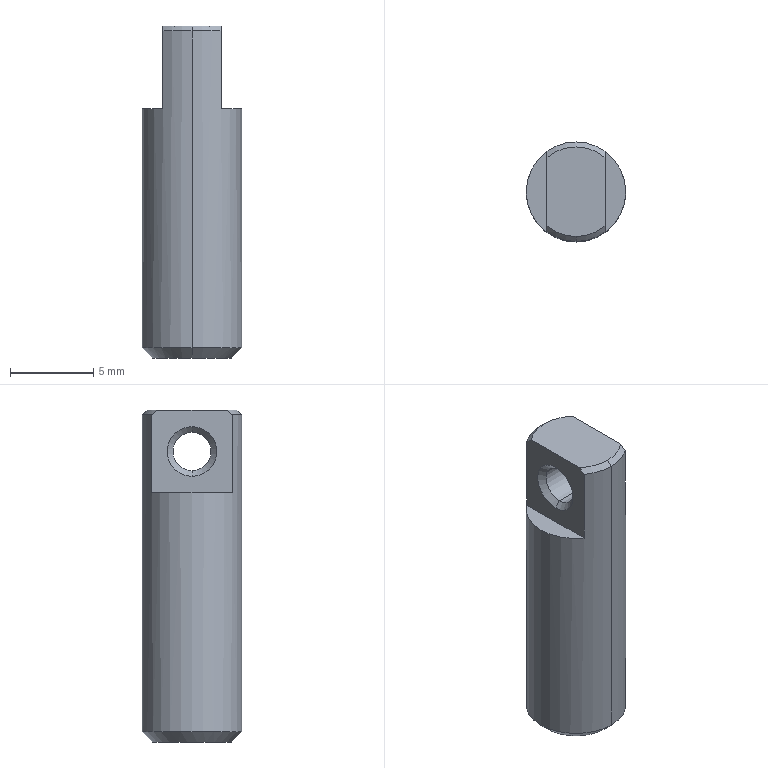Component | SolidWorks | SpringPillarFFE01-D6-L20-1 | 1 solid | 19 faces | box 6 x 6 x 20 mm | volume 504 mm3 | cone 9 | plane 6 | cylinder 4 | commonest cylinder face diameters 6 x2 2.3 x2 | material Purchased Part
STEP:
#1=CARTESIAN_POINT('',(-2.126,-0.315,-0.6845));
#2=VERTEX_POINT('',#1);
#3=CARTESIAN_POINT('',(-2.126,-0.5512,-0.6845));
#4=VERTEX_POINT('',#3);
#5=CARTESIAN_POINT('',(-2.126,-0.4331,-0.6845));
#6=DIRECTION('',(0.,0.,1.));
#7=DIRECTION('',(0.,1.,0.));
#8=AXIS2_PLACEMENT_3D('',#5,#6,#7);
#9=CIRCLE('',#8,0.1181);
#10=EDGE_CURVE('',#2,#4,#9,.T.);
#11=ORIENTED_EDGE('',*,*,#10,.T.);
#12=CARTESIAN_POINT('',(-2.126,-0.5512,0.06693));
#13=VERTEX_POINT('',#12);
#14=CARTESIAN_POINT('',(-2.126,-0.5512,-0.7087));
#15=DIRECTION('',(0.,0.,1.));
#16=VECTOR('',#15,39.37);
#17=LINE('',#14,#16);
#18=EDGE_CURVE('',#4,#13,#17,.T.);
#19=ORIENTED_EDGE('',*,*,#18,.T.);
#20=CARTESIAN_POINT('',(-2.195,-0.529,0.06693));
#21=VERTEX_POINT('',#20);
#22=CARTESIAN_POINT('',(-2.126,-0.4331,0.06693));
#23=DIRECTION('',(0.,0.,-1.));
#24=DIRECTION('',(0.,1.,0.));
#25=AXIS2_PLACEMENT_3D('',#22,#23,#24);
#26=CIRCLE('',#25,0.1181);
#27=EDGE_CURVE('',#13,#21,#26,.T.);
#28=ORIENTED_EDGE('',*,*,#27,.T.);
#29=CARTESIAN_POINT('',(-2.195,-0.529,-0.1181));
#30=VERTEX_POINT('',#29);
#31=CARTESIAN_POINT('',(-2.195,-0.529,-0.7087));
#32=DIRECTION('',(0.,0.,-1.));
#33=VECTOR('',#32,39.37);
#34=LINE('',#31,#33);
#35=EDGE_CURVE('',#21,#30,#34,.T.);
#36=ORIENTED_EDGE('',*,*,#35,.T.);
#37=CARTESIAN_POINT('',(-2.195,-0.3371,-0.1181));
#38=VERTEX_POINT('',#37);
#39=CARTESIAN_POINT('',(-2.126,-0.4331,-0.1181));
#40=DIRECTION('',(0.,0.,-1.));
#41=DIRECTION('',(0.,1.,0.));
#42=AXIS2_PLACEMENT_3D('',#39,#40,#41);
#43=CIRCLE('',#42,0.1181);
#44=EDGE_CURVE('',#30,#38,#43,.T.);
#45=ORIENTED_EDGE('',*,*,#44,.T.);
#46=CARTESIAN_POINT('',(-2.195,-0.3371,0.06693));
#47=VERTEX_POINT('',#46);
#48=CARTESIAN_POINT('',(-2.195,-0.3371,-0.7087));
#49=DIRECTION('',(0.,0.,1.));
#50=VECTOR('',#49,39.37);
#51=LINE('',#48,#50);
#52=EDGE_CURVE('',#38,#47,#51,.T.);
#53=ORIENTED_EDGE('',*,*,#52,.T.);
#54=CARTESIAN_POINT('',(-2.126,-0.315,0.06693));
#55=VERTEX_POINT('',#54);
#56=CARTESIAN_POINT('',(-2.126,-0.4331,0.06693));
#57=DIRECTION('',(0.,0.,-1.));
#58=DIRECTION('',(-0.,1.,0.));
#59=AXIS2_PLACEMENT_3D('',#56,#57,#58);
#60=CIRCLE('',#59,0.1181);
#61=EDGE_CURVE('',#47,#55,#60,.T.);
#62=ORIENTED_EDGE('',*,*,#61,.T.);
#63=CARTESIAN_POINT('',(-2.126,-0.315,-0.7087));
#64=DIRECTION('',(0.,0.,1.));
#65=VECTOR('',#64,39.37);
#66=LINE('',#63,#65);
#67=EDGE_CURVE('',#2,#55,#66,.T.);
#68=ORIENTED_EDGE('',*,*,#67,.F.);
#69=EDGE_LOOP('',(#11,#19,#28,#36,#45,#53,#62,#68));
#70=FACE_OUTER_BOUND('',#69,.T.);
#71=CARTESIAN_POINT('',(-2.126,-0.4331,-0.7087));
#72=DIRECTION('',(0.,0.,1.));
#73=DIRECTION('',(0.,1.,0.));
#74=AXIS2_PLACEMENT_3D('',#71,#72,#73);
#75=CYLINDRICAL_SURFACE('',#74,0.1181);
#76=ADVANCED_FACE('',(#70),#75,.T.);
#77=CARTESIAN_POINT('',(-2.057,-0.514,0.07874));
#78=VERTEX_POINT('',#77);
#79=CARTESIAN_POINT('',(-2.126,-0.5394,0.07874));
#80=VERTEX_POINT('',#79);
#81=CARTESIAN_POINT('',(-2.126,-0.4331,0.07874));
#82=DIRECTION('',(0.,0.,-1.));
#83=DIRECTION('',(0.,-1.,0.));
#84=AXIS2_PLACEMENT_3D('',#81,#82,#83);
#85=CIRCLE('',#84,0.1063);
#86=EDGE_CURVE('',#78,#80,#85,.T.);
#87=ORIENTED_EDGE('',*,*,#86,.T.);
#88=CARTESIAN_POINT('',(-2.126,-0.5512,0.06693));
#89=DIRECTION('',(0.,-0.7071,-0.7071));
#90=VECTOR('',#89,39.37);
#91=LINE('',#88,#90);
#92=EDGE_CURVE('',#80,#13,#91,.T.);
#93=ORIENTED_EDGE('',*,*,#92,.T.);
#94=CARTESIAN_POINT('',(-2.057,-0.529,0.06693));
#95=VERTEX_POINT('',#94);
#96=CARTESIAN_POINT('',(-2.126,-0.4331,0.06693));
#97=DIRECTION('',(0.,0.,-1.));
#98=DIRECTION('',(0.,1.,0.));
#99=AXIS2_PLACEMENT_3D('',#96,#97,#98);
#100=CIRCLE('',#99,0.1181);
#101=EDGE_CURVE('',#95,#13,#100,.T.);
#102=ORIENTED_EDGE('',*,*,#101,.F.);
#103=CARTESIAN_POINT('',(-2.057,-0.514,0.07874));
#104=CARTESIAN_POINT('',(-2.057,-0.5191,0.07489));
#105=CARTESIAN_POINT('',(-2.057,-0.5241,0.07094));
#106=CARTESIAN_POINT('',(-2.057,-0.529,0.06693));
#107=B_SPLINE_CURVE_WITH_KNOTS('',3,(#103,#104,#105,#106),.UNSPECIFIED.,.F.,.F.,(4,4),(0.,0.0004846),.UNSPECIFIED.);
#108=EDGE_CURVE('',#78,#95,#107,.T.);
#109=ORIENTED_EDGE('',*,*,#108,.F.);
#110=EDGE_LOOP('',(#87,#93,#102,#109));
#111=FACE_OUTER_BOUND('',#110,.T.);
#112=CARTESIAN_POINT('',(-2.126,-0.4331,0.06693));
#113=DIRECTION('',(0.,0.,-1.));
#114=DIRECTION('',(0.,-1.,0.));
#115=AXIS2_PLACEMENT_3D('',#112,#113,#114);
#116=CONICAL_SURFACE('',#115,0.1181,0.7854);
#117=ADVANCED_FACE('',(#111),#116,.T.);
#118=CARTESIAN_POINT('',(-2.126,-0.3391,-0.7087));
#119=VERTEX_POINT('',#118);
#120=CARTESIAN_POINT('',(-2.126,-0.527,-0.7087));
#121=VERTEX_POINT('',#120);
#122=CARTESIAN_POINT('',(-2.126,-0.4331,-0.7087));
#123=DIRECTION('',(0.,0.,1.));
#124=DIRECTION('',(0.,1.,0.));
#125=AXIS2_PLACEMENT_3D('',#122,#123,#124);
#126=CIRCLE('',#125,0.09396);
#127=EDGE_CURVE('',#119,#121,#126,.T.);
#128=ORIENTED_EDGE('',*,*,#127,.T.);
#129=CARTESIAN_POINT('',(-2.126,-0.5512,-0.6845));
#130=DIRECTION('',(-0.,-0.7071,0.7071));
#131=VECTOR('',#130,39.37);
#132=LINE('',#129,#131);
#133=EDGE_CURVE('',#121,#4,#132,.T.);
#134=ORIENTED_EDGE('',*,*,#133,.T.);
#135=ORIENTED_EDGE('',*,*,#10,.F.);
#136=CARTESIAN_POINT('',(-2.126,-0.315,-0.6845));
#137=DIRECTION('',(0.,0.7071,0.7071));
#138=VECTOR('',#137,39.37);
#139=LINE('',#136,#138);
#140=EDGE_CURVE('',#119,#2,#139,.T.);
#141=ORIENTED_EDGE('',*,*,#140,.F.);
#142=EDGE_LOOP('',(#128,#134,#135,#141));
#143=FACE_OUTER_BOUND('',#142,.T.);
#144=CARTESIAN_POINT('',(-2.126,-0.4331,-0.6845));
#145=DIRECTION('',(0.,0.,1.));
#146=DIRECTION('',(0.,1.,0.));
#147=AXIS2_PLACEMENT_3D('',#144,#145,#146);
#148=CONICAL_SURFACE('',#147,0.1181,0.7854);
#149=ADVANCED_FACE('',(#143),#148,.T.);
#150=CARTESIAN_POINT('',(-2.071,-0.4331,0.02559));
#151=VERTEX_POINT('',#150);
#152=CARTESIAN_POINT('',(-2.071,-0.4331,-0.06496));
#153=VERTEX_POINT('',#152);
#154=CARTESIAN_POINT('',(-2.071,-0.4331,-0.01969));
#155=DIRECTION('',(1.,0.,0.));
#156=DIRECTION('',(0.,0.,-1.));
#157=AXIS2_PLACEMENT_3D('',#154,#155,#156);
#158=CIRCLE('',#157,0.04528);
#159=EDGE_CURVE('',#151,#153,#158,.T.);
#160=ORIENTED_EDGE('',*,*,#159,.F.);
#161=CARTESIAN_POINT('',(-2.057,-0.4331,0.03937));
#162=VERTEX_POINT('',#161);
#163=CARTESIAN_POINT('',(-2.057,-0.4331,0.03937));
#164=DIRECTION('',(0.7071,0.,0.7071));
#165=VECTOR('',#164,39.37);
#166=LINE('',#163,#165);
#167=EDGE_CURVE('',#151,#162,#166,.T.);
#168=ORIENTED_EDGE('',*,*,#167,.T.);
#169=CARTESIAN_POINT('',(-2.057,-0.4331,-0.07874));
#170=VERTEX_POINT('',#169);
#171=CARTESIAN_POINT('',(-2.057,-0.4331,-0.01969));
#172=DIRECTION('',(-1.,0.,0.));
#173=DIRECTION('',(0.,0.,-1.));
#174=AXIS2_PLACEMENT_3D('',#171,#172,#173);
#175=CIRCLE('',#174,0.05906);
#176=EDGE_CURVE('',#170,#162,#175,.T.);
#177=ORIENTED_EDGE('',*,*,#176,.F.);
#178=CARTESIAN_POINT('',(-2.057,-0.4331,-0.07874));
#179=DIRECTION('',(0.7071,0.,-0.7071));
#180=VECTOR('',#179,39.37);
#181=LINE('',#178,#180);
#182=EDGE_CURVE('',#153,#170,#181,.T.);
#183=ORIENTED_EDGE('',*,*,#182,.F.);
#184=EDGE_LOOP('',(#160,#168,#177,#183));
#185=FACE_OUTER_BOUND('',#184,.T.);
#186=CARTESIAN_POINT('',(-2.057,-0.4331,-0.01969));
#187=DIRECTION('',(1.,0.,0.));
#188=DIRECTION('',(0.,0.,-1.));
#189=AXIS2_PLACEMENT_3D('',#186,#187,#188);
#190=CONICAL_SURFACE('',#189,0.05906,0.7854);
#191=ADVANCED_FACE('',(#185),#190,.F.);
#192=CARTESIAN_POINT('',(-2.181,-0.4331,-0.06496));
#193=VERTEX_POINT('',#192);
#194=CARTESIAN_POINT('',(-2.181,-0.4331,0.02559));
#195=VERTEX_POINT('',#194);
#196=CARTESIAN_POINT('',(-2.181,-0.4331,-0.01969));
#197=DIRECTION('',(-1.,0.,0.));
#198=DIRECTION('',(0.,0.,1.));
#199=AXIS2_PLACEMENT_3D('',#196,#197,#198);
#200=CIRCLE('',#199,0.04528);
#201=EDGE_CURVE('',#193,#195,#200,.T.);
#202=ORIENTED_EDGE('',*,*,#201,.F.);
#203=CARTESIAN_POINT('',(-2.195,-0.4331,-0.07874));
#204=VERTEX_POINT('',#203);
#205=CARTESIAN_POINT('',(-2.195,-0.4331,-0.07874));
#206=DIRECTION('',(-0.7071,0.,-0.7071));
#207=VECTOR('',#206,39.37);
#208=LINE('',#205,#207);
#209=EDGE_CURVE('',#193,#204,#208,.T.);
#210=ORIENTED_EDGE('',*,*,#209,.T.);
#211=CARTESIAN_POINT('',(-2.195,-0.4331,0.03937));
#212=VERTEX_POINT('',#211);
#213=CARTESIAN_POINT('',(-2.195,-0.4331,-0.01969));
#214=DIRECTION('',(1.,0.,0.));
#215=DIRECTION('',(0.,0.,1.));
#216=AXIS2_PLACEMENT_3D('',#213,#214,#215);
#217=CIRCLE('',#216,0.05906);
#218=EDGE_CURVE('',#212,#204,#217,.T.);
#219=ORIENTED_EDGE('',*,*,#218,.F.);
#220=CARTESIAN_POINT('',(-2.195,-0.4331,0.03937));
#221=DIRECTION('',(-0.7071,0.,0.7071));
#222=VECTOR('',#221,39.37);
#223=LINE('',#220,#222);
#224=EDGE_CURVE('',#195,#212,#223,.T.);
#225=ORIENTED_EDGE('',*,*,#224,.F.);
#226=EDGE_LOOP('',(#202,#210,#219,#225));
#227=FACE_OUTER_BOUND('',#226,.T.);
#228=CARTESIAN_POINT('',(-2.195,-0.4331,-0.01969));
#229=DIRECTION('',(-1.,0.,0.));
#230=DIRECTION('',(0.,0.,1.));
#231=AXIS2_PLACEMENT_3D('',#228,#229,#230);
#232=CONICAL_SURFACE('',#231,0.05906,0.7854);
#233=ADVANCED_FACE('',(#227),#232,.F.);
#234=ORIENTED_EDGE('',*,*,#159,.T.);
#235=CARTESIAN_POINT('',(-2.057,-0.4331,-0.06496));
#236=DIRECTION('',(-1.,0.,0.));
#237=VECTOR('',#236,39.37);
#238=LINE('',#235,#237);
#239=EDGE_CURVE('',#153,#193,#238,.T.);
#240=ORIENTED_EDGE('',*,*,#239,.T.);
#241=ORIENTED_EDGE('',*,*,#201,.T.);
#242=CARTESIAN_POINT('',(-2.057,-0.4331,0.02559));
#243=DIRECTION('',(-1.,0.,0.));
#244=VECTOR('',#243,39.37);
#245=LINE('',#242,#244);
#246=EDGE_CURVE('',#151,#195,#245,.T.);
#247=ORIENTED_EDGE('',*,*,#246,.F.);
#248=EDGE_LOOP('',(#234,#240,#241,#247));
#249=FACE_OUTER_BOUND('',#248,.T.);
#250=CARTESIAN_POINT('',(-2.057,-0.4331,-0.01969));
#251=DIRECTION('',(-1.,0.,0.));
#252=DIRECTION('',(0.,0.,1.));
#253=AXIS2_PLACEMENT_3D('',#250,#251,#252);
#254=CYLINDRICAL_SURFACE('',#253,0.04528);
#255=ADVANCED_FACE('',(#249),#254,.F.);
#256=ORIENTED_EDGE('',*,*,#18,.F.);
#257=CARTESIAN_POINT('',(-2.126,-0.4331,-0.6845));
#258=DIRECTION('',(0.,0.,1.));
#259=DIRECTION('',(0.,1.,0.));
#260=AXIS2_PLACEMENT_3D('',#257,#258,#259);
#261=CIRCLE('',#260,0.1181);
#262=EDGE_CURVE('',#4,#2,#261,.T.);
#263=ORIENTED_EDGE('',*,*,#262,.T.);
#264=ORIENTED_EDGE('',*,*,#67,.T.);
#265=CARTESIAN_POINT('',(-2.057,-0.3371,0.06693));
#266=VERTEX_POINT('',#265);
#267=CARTESIAN_POINT('',(-2.126,-0.4331,0.06693));
#268=DIRECTION('',(0.,0.,-1.));
#269=DIRECTION('',(0.,1.,0.));
#270=AXIS2_PLACEMENT_3D('',#267,#268,#269);
#271=CIRCLE('',#270,0.1181);
#272=EDGE_CURVE('',#55,#266,#271,.T.);
#273=ORIENTED_EDGE('',*,*,#272,.T.);
#274=CARTESIAN_POINT('',(-2.057,-0.3371,-0.1181));
#275=VERTEX_POINT('',#274);
#276=CARTESIAN_POINT('',(-2.057,-0.3371,-0.7087));
#277=DIRECTION('',(0.,0.,-1.));
#278=VECTOR('',#277,39.37);
#279=LINE('',#276,#278);
#280=EDGE_CURVE('',#266,#275,#279,.T.);
#281=ORIENTED_EDGE('',*,*,#280,.T.);
#282=CARTESIAN_POINT('',(-2.057,-0.529,-0.1181));
#283=VERTEX_POINT('',#282);
#284=CARTESIAN_POINT('',(-2.126,-0.4331,-0.1181));
#285=DIRECTION('',(0.,0.,-1.));
#286=DIRECTION('',(0.,1.,0.));
#287=AXIS2_PLACEMENT_3D('',#284,#285,#286);
#288=CIRCLE('',#287,0.1181);
#289=EDGE_CURVE('',#275,#283,#288,.T.);
#290=ORIENTED_EDGE('',*,*,#289,.T.);
#291=CARTESIAN_POINT('',(-2.057,-0.529,-0.7087));
#292=DIRECTION('',(0.,0.,1.));
#293=VECTOR('',#292,39.37);
#294=LINE('',#291,#293);
#295=EDGE_CURVE('',#283,#95,#294,.T.);
#296=ORIENTED_EDGE('',*,*,#295,.T.);
#297=ORIENTED_EDGE('',*,*,#101,.T.);
#298=EDGE_LOOP('',(#256,#263,#264,#273,#281,#290,#296,#297));
#299=FACE_OUTER_BOUND('',#298,.T.);
#300=CARTESIAN_POINT('',(-2.126,-0.4331,-0.7087));
#301=DIRECTION('',(0.,0.,1.));
#302=DIRECTION('',(0.,1.,0.));
#303=AXIS2_PLACEMENT_3D('',#300,#301,#302);
#304=CYLINDRICAL_SURFACE('',#303,0.1181);
#305=ADVANCED_FACE('',(#299),#304,.T.);
#306=CARTESIAN_POINT('',(-2.057,-0.315,-0.1181));
#307=DIRECTION('',(0.,-1.,0.));
#308=VECTOR('',#307,39.37);
#309=LINE('',#306,#308);
#310=EDGE_CURVE('',#275,#283,#309,.T.);
#311=ORIENTED_EDGE('',*,*,#310,.T.);
#312=ORIENTED_EDGE('',*,*,#289,.F.);
#313=EDGE_LOOP('',(#311,#312));
#314=FACE_OUTER_BOUND('',#313,.T.);
#315=CARTESIAN_POINT('',(-2.008,-0.315,-0.1181));
#316=DIRECTION('',(0.,0.,1.));
#317=DIRECTION('',(0.,1.,0.));
#318=AXIS2_PLACEMENT_3D('',#315,#316,#317);
#319=PLANE('',#318);
#320=ADVANCED_FACE('',(#314),#319,.T.);
#321=ORIENTED_EDGE('',*,*,#176,.T.);
#322=CARTESIAN_POINT('',(-2.057,-0.4331,-0.01969));
#323=DIRECTION('',(-1.,0.,0.));
#324=DIRECTION('',(0.,0.,-1.));
#325=AXIS2_PLACEMENT_3D('',#322,#323,#324);
#326=CIRCLE('',#325,0.05906);
#327=EDGE_CURVE('',#162,#170,#326,.T.);
#328=ORIENTED_EDGE('',*,*,#327,.T.);
#329=EDGE_LOOP('',(#321,#328));
#330=FACE_BOUND('',#329,.T.);
#331=CARTESIAN_POINT('',(-2.057,-0.3521,0.07874));
#332=VERTEX_POINT('',#331);
#333=CARTESIAN_POINT('',(-2.057,-0.3371,0.06693));
#334=CARTESIAN_POINT('',(-2.057,-0.3421,0.07094));
#335=CARTESIAN_POINT('',(-2.057,-0.3471,0.07489));
#336=CARTESIAN_POINT('',(-2.057,-0.3521,0.07874));
#337=B_SPLINE_CURVE_WITH_KNOTS('',3,(#333,#334,#335,#336),.UNSPECIFIED.,.F.,.F.,(4,4),(0.,0.0004846),.UNSPECIFIED.);
#338=EDGE_CURVE('',#266,#332,#337,.T.);
#339=ORIENTED_EDGE('',*,*,#338,.T.);
#340=CARTESIAN_POINT('',(-2.057,-0.315,0.07874));
#341=DIRECTION('',(0.,-1.,0.));
#342=VECTOR('',#341,39.37);
#343=LINE('',#340,#342);
#344=EDGE_CURVE('',#332,#78,#343,.T.);
#345=ORIENTED_EDGE('',*,*,#344,.T.);
#346=ORIENTED_EDGE('',*,*,#108,.T.);
#347=ORIENTED_EDGE('',*,*,#295,.F.);
#348=ORIENTED_EDGE('',*,*,#310,.F.);
#349=ORIENTED_EDGE('',*,*,#280,.F.);
#350=EDGE_LOOP('',(#339,#345,#346,#347,#348,#349));
#351=FACE_OUTER_BOUND('',#350,.T.);
#352=CARTESIAN_POINT('',(-2.057,-0.315,-0.1181));
#353=DIRECTION('',(1.,0.,0.));
#354=DIRECTION('',(0.,0.,-1.));
#355=AXIS2_PLACEMENT_3D('',#352,#353,#354);
#356=PLANE('',#355);
#357=ADVANCED_FACE('',(#330,#351),#356,.T.);
#358=CARTESIAN_POINT('',(-2.195,-0.3521,0.07874));
#359=VERTEX_POINT('',#358);
#360=CARTESIAN_POINT('',(-2.195,-0.3371,0.06693));
#361=CARTESIAN_POINT('',(-2.195,-0.3421,0.07094));
#362=CARTESIAN_POINT('',(-2.195,-0.3471,0.07489));
#363=CARTESIAN_POINT('',(-2.195,-0.3521,0.07874));
#364=B_SPLINE_CURVE_WITH_KNOTS('',3,(#360,#361,#362,#363),.UNSPECIFIED.,.F.,.F.,(4,4),(0.,0.0004846),.UNSPECIFIED.);
#365=EDGE_CURVE('',#47,#359,#364,.T.);
#366=ORIENTED_EDGE('',*,*,#365,.T.);
#367=CARTESIAN_POINT('',(-2.126,-0.4331,0.07874));
#368=DIRECTION('',(0.,0.,-1.));
#369=DIRECTION('',(0.,-1.,0.));
#370=AXIS2_PLACEMENT_3D('',#367,#368,#369);
#371=CIRCLE('',#370,0.1063);
#372=EDGE_CURVE('',#359,#332,#371,.T.);
#373=ORIENTED_EDGE('',*,*,#372,.T.);
#374=ORIENTED_EDGE('',*,*,#338,.F.);
#375=ORIENTED_EDGE('',*,*,#272,.F.);
#376=ORIENTED_EDGE('',*,*,#61,.F.);
#377=EDGE_LOOP('',(#366,#373,#374,#375,#376));
#378=FACE_OUTER_BOUND('',#377,.T.);
#379=CARTESIAN_POINT('',(-2.126,-0.4331,0.06693));
#380=DIRECTION('',(0.,0.,-1.));
#381=DIRECTION('',(0.,-1.,0.));
#382=AXIS2_PLACEMENT_3D('',#379,#380,#381);
#383=CONICAL_SURFACE('',#382,0.1181,0.7854);
#384=ADVANCED_FACE('',(#378),#383,.T.);
#385=ORIENTED_EDGE('',*,*,#218,.T.);
#386=CARTESIAN_POINT('',(-2.195,-0.4331,-0.01969));
#387=DIRECTION('',(1.,0.,0.));
#388=DIRECTION('',(0.,0.,1.));
#389=AXIS2_PLACEMENT_3D('',#386,#387,#388);
#390=CIRCLE('',#389,0.05906);
#391=EDGE_CURVE('',#204,#212,#390,.T.);
#392=ORIENTED_EDGE('',*,*,#391,.T.);
#393=EDGE_LOOP('',(#385,#392));
#394=FACE_BOUND('',#393,.T.);
#395=CARTESIAN_POINT('',(-2.195,-0.514,0.07874));
#396=VERTEX_POINT('',#395);
#397=CARTESIAN_POINT('',(-2.195,-0.529,0.06693));
#398=CARTESIAN_POINT('',(-2.195,-0.5241,0.07094));
#399=CARTESIAN_POINT('',(-2.195,-0.5191,0.07489));
#400=CARTESIAN_POINT('',(-2.195,-0.514,0.07874));
#401=B_SPLINE_CURVE_WITH_KNOTS('',3,(#397,#398,#399,#400),.UNSPECIFIED.,.F.,.F.,(4,4),(0.,0.0004846),.UNSPECIFIED.);
#402=EDGE_CURVE('',#21,#396,#401,.T.);
#403=ORIENTED_EDGE('',*,*,#402,.T.);
#404=CARTESIAN_POINT('',(-2.195,-0.315,0.07874));
#405=DIRECTION('',(0.,1.,0.));
#406=VECTOR('',#405,39.37);
#407=LINE('',#404,#406);
#408=EDGE_CURVE('',#396,#359,#407,.T.);
#409=ORIENTED_EDGE('',*,*,#408,.T.);
#410=ORIENTED_EDGE('',*,*,#365,.F.);
#411=ORIENTED_EDGE('',*,*,#52,.F.);
#412=CARTESIAN_POINT('',(-2.195,-0.315,-0.1181));
#413=DIRECTION('',(0.,-1.,0.));
#414=VECTOR('',#413,39.37);
#415=LINE('',#412,#414);
#416=EDGE_CURVE('',#38,#30,#415,.T.);
#417=ORIENTED_EDGE('',*,*,#416,.T.);
#418=ORIENTED_EDGE('',*,*,#35,.F.);
#419=EDGE_LOOP('',(#403,#409,#410,#411,#417,#418));
#420=FACE_OUTER_BOUND('',#419,.T.);
#421=CARTESIAN_POINT('',(-2.195,-0.315,0.07874));
#422=DIRECTION('',(-1.,0.,0.));
#423=DIRECTION('',(0.,0.,1.));
#424=AXIS2_PLACEMENT_3D('',#421,#422,#423);
#425=PLANE('',#424);
#426=ADVANCED_FACE('',(#394,#420),#425,.T.);
#427=ORIENTED_EDGE('',*,*,#416,.F.);
#428=ORIENTED_EDGE('',*,*,#44,.F.);
#429=EDGE_LOOP('',(#427,#428));
#430=FACE_OUTER_BOUND('',#429,.T.);
#431=CARTESIAN_POINT('',(-2.195,-0.315,-0.1181));
#432=DIRECTION('',(0.,0.,1.));
#433=DIRECTION('',(0.,1.,0.));
#434=AXIS2_PLACEMENT_3D('',#431,#432,#433);
#435=PLANE('',#434);
#436=ADVANCED_FACE('',(#430),#435,.T.);
#437=ORIENTED_EDGE('',*,*,#92,.F.);
#438=CARTESIAN_POINT('',(-2.126,-0.4331,0.07874));
#439=DIRECTION('',(0.,0.,-1.));
#440=DIRECTION('',(0.,-1.,0.));
#441=AXIS2_PLACEMENT_3D('',#438,#439,#440);
#442=CIRCLE('',#441,0.1063);
#443=EDGE_CURVE('',#80,#396,#442,.T.);
#444=ORIENTED_EDGE('',*,*,#443,.T.);
#445=ORIENTED_EDGE('',*,*,#402,.F.);
#446=ORIENTED_EDGE('',*,*,#27,.F.);
#447=EDGE_LOOP('',(#437,#444,#445,#446));
#448=FACE_OUTER_BOUND('',#447,.T.);
#449=CARTESIAN_POINT('',(-2.126,-0.4331,0.06693));
#450=DIRECTION('',(0.,0.,-1.));
#451=DIRECTION('',(0.,-1.,0.));
#452=AXIS2_PLACEMENT_3D('',#449,#450,#451);
#453=CONICAL_SURFACE('',#452,0.1181,0.7854);
#454=ADVANCED_FACE('',(#448),#453,.T.);
#455=ORIENTED_EDGE('',*,*,#133,.F.);
#456=CARTESIAN_POINT('',(-2.126,-0.4331,-0.7087));
#457=DIRECTION('',(0.,0.,1.));
#458=DIRECTION('',(0.,1.,0.));
#459=AXIS2_PLACEMENT_3D('',#456,#457,#458);
#460=CIRCLE('',#459,0.09396);
#461=EDGE_CURVE('',#121,#119,#460,.T.);
#462=ORIENTED_EDGE('',*,*,#461,.T.);
#463=ORIENTED_EDGE('',*,*,#140,.T.);
#464=ORIENTED_EDGE('',*,*,#262,.F.);
#465=EDGE_LOOP('',(#455,#462,#463,#464));
#466=FACE_OUTER_BOUND('',#465,.T.);
#467=CARTESIAN_POINT('',(-2.126,-0.4331,-0.6845));
#468=DIRECTION('',(0.,0.,1.));
#469=DIRECTION('',(0.,1.,0.));
#470=AXIS2_PLACEMENT_3D('',#467,#468,#469);
#471=CONICAL_SURFACE('',#470,0.1181,0.7854);
#472=ADVANCED_FACE('',(#466),#471,.T.);
#473=ORIENTED_EDGE('',*,*,#167,.F.);
#474=CARTESIAN_POINT('',(-2.071,-0.4331,-0.01969));
#475=DIRECTION('',(1.,0.,0.));
#476=DIRECTION('',(0.,0.,-1.));
#477=AXIS2_PLACEMENT_3D('',#474,#475,#476);
#478=CIRCLE('',#477,0.04528);
#479=EDGE_CURVE('',#153,#151,#478,.T.);
#480=ORIENTED_EDGE('',*,*,#479,.F.);
#481=ORIENTED_EDGE('',*,*,#182,.T.);
#482=ORIENTED_EDGE('',*,*,#327,.F.);
#483=EDGE_LOOP('',(#473,#480,#481,#482));
#484=FACE_OUTER_BOUND('',#483,.T.);
#485=CARTESIAN_POINT('',(-2.057,-0.4331,-0.01969));
#486=DIRECTION('',(1.,0.,0.));
#487=DIRECTION('',(0.,0.,-1.));
#488=AXIS2_PLACEMENT_3D('',#485,#486,#487);
#489=CONICAL_SURFACE('',#488,0.05906,0.7854);
#490=ADVANCED_FACE('',(#484),#489,.F.);
#491=ORIENTED_EDGE('',*,*,#86,.F.);
#492=ORIENTED_EDGE('',*,*,#344,.F.);
#493=ORIENTED_EDGE('',*,*,#372,.F.);
#494=ORIENTED_EDGE('',*,*,#408,.F.);
#495=ORIENTED_EDGE('',*,*,#443,.F.);
#496=EDGE_LOOP('',(#491,#492,#493,#494,#495));
#497=FACE_OUTER_BOUND('',#496,.T.);
#498=CARTESIAN_POINT('',(-2.126,-0.4331,0.07874));
#499=DIRECTION('',(0.,0.,-1.));
#500=DIRECTION('',(0.,-1.,0.));
#501=AXIS2_PLACEMENT_3D('',#498,#499,#500);
#502=PLANE('',#501);
#503=ADVANCED_FACE('',(#497),#502,.F.);
#504=ORIENTED_EDGE('',*,*,#209,.F.);
#505=CARTESIAN_POINT('',(-2.181,-0.4331,-0.01969));
#506=DIRECTION('',(-1.,0.,0.));
#507=DIRECTION('',(0.,0.,1.));
#508=AXIS2_PLACEMENT_3D('',#505,#506,#507);
#509=CIRCLE('',#508,0.04528);
#510=EDGE_CURVE('',#195,#193,#509,.T.);
#511=ORIENTED_EDGE('',*,*,#510,.F.);
#512=ORIENTED_EDGE('',*,*,#224,.T.);
#513=ORIENTED_EDGE('',*,*,#391,.F.);
#514=EDGE_LOOP('',(#504,#511,#512,#513));
#515=FACE_OUTER_BOUND('',#514,.T.);
#516=CARTESIAN_POINT('',(-2.195,-0.4331,-0.01969));
#517=DIRECTION('',(-1.,0.,0.));
#518=DIRECTION('',(0.,0.,1.));
#519=AXIS2_PLACEMENT_3D('',#516,#517,#518);
#520=CONICAL_SURFACE('',#519,0.05906,0.7854);
#521=ADVANCED_FACE('',(#515),#520,.F.);
#522=ORIENTED_EDGE('',*,*,#127,.F.);
#523=ORIENTED_EDGE('',*,*,#461,.F.);
#524=EDGE_LOOP('',(#522,#523));
#525=FACE_OUTER_BOUND('',#524,.T.);
#526=CARTESIAN_POINT('',(-2.22,-0.4331,-0.7087));
#527=DIRECTION('',(0.,0.,1.));
#528=DIRECTION('',(0.,1.,0.));
#529=AXIS2_PLACEMENT_3D('',#526,#527,#528);
#530=PLANE('',#529);
#531=ADVANCED_FACE('',(#525),#530,.F.);
#532=ORIENTED_EDGE('',*,*,#239,.F.);
#533=ORIENTED_EDGE('',*,*,#479,.T.);
#534=ORIENTED_EDGE('',*,*,#246,.T.);
#535=ORIENTED_EDGE('',*,*,#510,.T.);
#536=EDGE_LOOP('',(#532,#533,#534,#535));
#537=FACE_OUTER_BOUND('',#536,.T.);
#538=CARTESIAN_POINT('',(-2.057,-0.4331,-0.01969));
#539=DIRECTION('',(-1.,0.,0.));
#540=DIRECTION('',(0.,0.,1.));
#541=AXIS2_PLACEMENT_3D('',#538,#539,#540);
#542=CYLINDRICAL_SURFACE('',#541,0.04528);
#543=ADVANCED_FACE('',(#537),#542,.F.);
#544=CLOSED_SHELL('',(#76,#117,#149,#191,#233,#255,#305,#320,#357,#384,#426,#436,#454,#472,#490,#503,#521,#531,#543));
#545=MANIFOLD_SOLID_BREP('',#544);
#546=CARTESIAN_POINT('',(0.,0.,0.));
#547=DIRECTION('',(0.,0.,1.));
#548=DIRECTION('',(1.,0.,0.));
#549=AXIS2_PLACEMENT_3D('',#546,#547,#548);
#550=(LENGTH_UNIT()NAMED_UNIT(*)SI_UNIT($,.METRE.));
#551=LENGTH_MEASURE_WITH_UNIT(LENGTH_MEASURE(0.0254),#550);
#552=DIMENSIONAL_EXPONENTS(1.,0.,0.,0.,0.,0.,0.);
#553=(CONVERSION_BASED_UNIT('',#551)LENGTH_UNIT()NAMED_UNIT(#552));
#554=UNCERTAINTY_MEASURE_WITH_UNIT(LENGTH_MEASURE(0.00001),#553,'','');
#555=(NAMED_UNIT(*)PLANE_ANGLE_UNIT()SI_UNIT($,.RADIAN.));
#556=(NAMED_UNIT(*)SI_UNIT($,.STERADIAN.)SOLID_ANGLE_UNIT());
#557=(GEOMETRIC_REPRESENTATION_CONTEXT(3)GLOBAL_UNCERTAINTY_ASSIGNED_CONTEXT((#554))GLOBAL_UNIT_ASSIGNED_CONTEXT((#553,#555,#556))REPRESENTATION_CONTEXT('',''));
#558=ADVANCED_BREP_SHAPE_REPRESENTATION('',(#545,#549),#557);
#559=COLOUR_RGB('',0.7922,0.8196,0.9333);
#560=FILL_AREA_STYLE_COLOUR('',#559);
#561=FILL_AREA_STYLE('',(#560));
#562=SURFACE_STYLE_FILL_AREA(#561);
#563=SURFACE_SIDE_STYLE('',(#562));
#564=SURFACE_STYLE_USAGE(.BOTH.,#563);
#565=PRESENTATION_STYLE_ASSIGNMENT((#564));
#566=STYLED_ITEM('',(#565),#545);
#567=(LENGTH_UNIT()NAMED_UNIT(*)SI_UNIT($,.METRE.));
#568=LENGTH_MEASURE_WITH_UNIT(LENGTH_MEASURE(0.0254),#567);
#569=DIMENSIONAL_EXPONENTS(1.,0.,0.,0.,0.,0.,0.);
#570=(CONVERSION_BASED_UNIT('',#568)LENGTH_UNIT()NAMED_UNIT(#569));
#571=UNCERTAINTY_MEASURE_WITH_UNIT(LENGTH_MEASURE(0.00001),#570,'','');
#572=(NAMED_UNIT(*)PLANE_ANGLE_UNIT()SI_UNIT($,.RADIAN.));
#573=(NAMED_UNIT(*)SI_UNIT($,.STERADIAN.)SOLID_ANGLE_UNIT());
#574=(GEOMETRIC_REPRESENTATION_CONTEXT(3)GLOBAL_UNCERTAINTY_ASSIGNED_CONTEXT((#571))GLOBAL_UNIT_ASSIGNED_CONTEXT((#570,#572,#573))REPRESENTATION_CONTEXT('',''));
#575=MECHANICAL_DESIGN_GEOMETRIC_PRESENTATION_REPRESENTATION('',(#566),#574);
#576=PRESENTATION_LAYER_ASSIGNMENT('','',(#566));